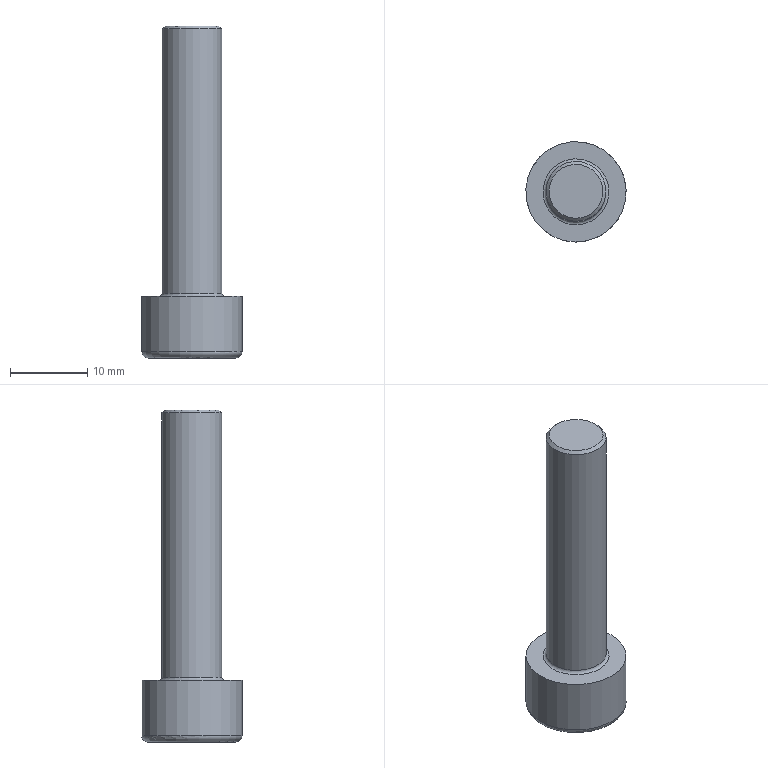Component | NX | GB-T70_1-2000_M8X35 | 1 solid | 27 faces | volume 2547 mm3 | plane 15 | cone 8 | cylinder 2 | torus 2 | commonest cylinder face diameters 7.76 x1 13 x1